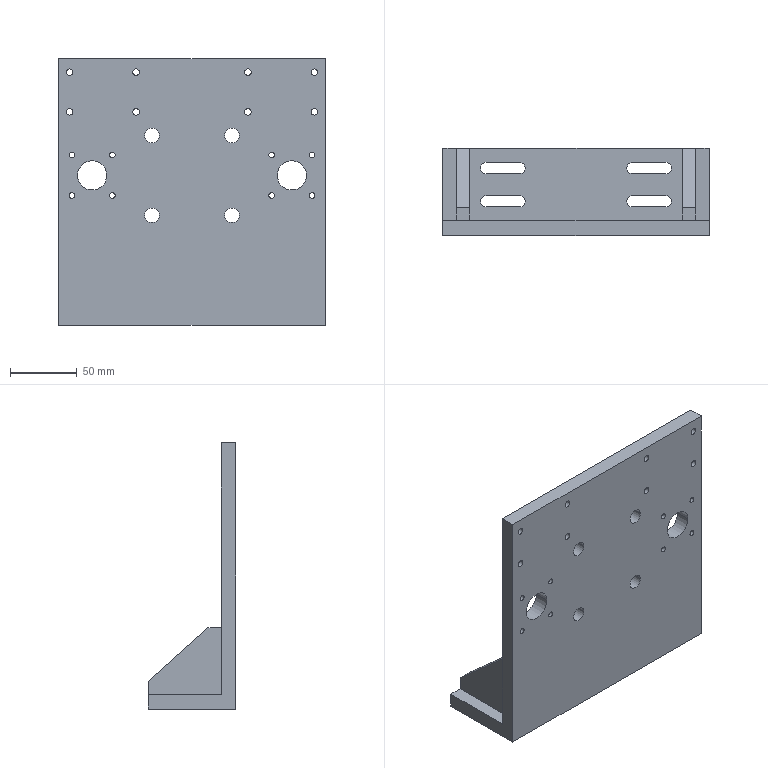Component | SolidWorks | YS01-053FixedBracket2-1 | 1 solid | 78 faces | box 200 x 66 x 200 mm | volume 570662 mm3 | cylinder 52 | plane 26 | commonest cylinder face diameters 5 x16 4.2 x16 11 x8 8.5 x8 22 x4
build123d program:
from build123d import *

# Parameters (mm, degrees)
SKETCH1_W                      = 200
SKETCH1_H                      = 200
BOSS_EXTRUDE1_DEPTH            = 11
SKETCH2_R                      = 11
CUT_EXTRUDE1_DEPTH             = 151.921
M5_TAPPED_HOLE1_AT_2_COUNT     = 2
M5_TAPPED_HOLE1_AT_2_PITCH     = 30.406
M5_TAPPED_HOLE1_AT_3_COUNT     = 2
M5_TAPPED_HOLE1_AT_3_PITCH     = 30.406
M5_TAPPED_HOLE1_AT_4_COUNT     = 2
M5_TAPPED_HOLE1_AT_4_PITCH     = 43
F_11_0_11_DIAMETER_HOLE2_D     = 11
F_11_0_11_DIAMETER_HOLE2_DEPTH = 14
F_11_0_11_DIAMETER_HOLE2_TIP   = 3.175
SKETCH7_W                      = 200
SKETCH7_H                      = 11
BOSS_EXTRUDE2_DEPTH            = 55
BOSS_EXTRUDE3_DEPTH            = 10
M6_TAPPED_HOLE1_AT_2_COUNT     = 2
M6_TAPPED_HOLE1_AT_2_PITCH     = 29.8
M6_TAPPED_HOLE1_AT_3_COUNT     = 2
M6_TAPPED_HOLE1_AT_3_PITCH     = 50
M6_TAPPED_HOLE1_AT_4_COUNT     = 2
M6_TAPPED_HOLE1_AT_4_PITCH     = 58.207
CUT_EXTRUDE2_DEPTH             = 224.779


with BuildPart() as part:
    # Sketch1 → Boss-Extrude1 (new body)
    with BuildSketch(Plane.XY):
        with Locations((0, -12.5)):
            Rectangle(SKETCH1_W, SKETCH1_H)
    extrude(amount=BOSS_EXTRUDE1_DEPTH)

    # Sketch2 → Cut-Extrude1 (cut, through all)
    with BuildSketch(Plane.XY.offset(11)):
        with Locations((75, 0)):
            Circle(SKETCH2_R)
        with Locations((-75, 0)):
            Circle(SKETCH2_R)
    extrude(amount=-CUT_EXTRUDE1_DEPTH, mode=Mode.SUBTRACT)

    # Sketch3 → M5 Tapped Hole1 (revolve, cut)
    with BuildSketch(Plane(origin=(90.203, 15.203, 0), x_dir=(0, 1, 0), z_dir=(1, 0, 0))):
        Polygon((0, 0), (0, 13.662), (2.1, 12.4), (2.1, 0), align=None)
    m5_tapped_hole1 = revolve(axis=Axis((90.203, 15.203, -6.35), (0, 0, 1)), mode=Mode.SUBTRACT)

    # M5 Tapped Hole1 at 2: M5 Tapped Hole1 ×2
    with Locations(*[(0, -i * M5_TAPPED_HOLE1_AT_2_PITCH, 0) for i in range(1, M5_TAPPED_HOLE1_AT_2_COUNT)]):
        add(m5_tapped_hole1, mode=Mode.SUBTRACT)

    # M5 Tapped Hole1 at 3: M5 Tapped Hole1 ×2
    with Locations(*[(-i * M5_TAPPED_HOLE1_AT_3_PITCH, 0, 0) for i in range(1, M5_TAPPED_HOLE1_AT_3_COUNT)]):
        add(m5_tapped_hole1, mode=Mode.SUBTRACT)

    # M5 Tapped Hole1 at 4: M5 Tapped Hole1 ×2
    with Locations(*[Vector(-0.7071, -0.7071, 0) * (i * M5_TAPPED_HOLE1_AT_4_PITCH) for i in range(1, M5_TAPPED_HOLE1_AT_4_COUNT)]):
        add(m5_tapped_hole1, mode=Mode.SUBTRACT)

    # Mirror1: M5 Tapped Hole1 across plane
    add(m5_tapped_hole1.mirror(Plane(origin=(0, 0, 0), x_dir=(0, 0, 1), z_dir=(1, 0, 0))), mode=Mode.SUBTRACT)

    # Mirror1 copy 1 sketch → Mirror1 copy 1 (revolve, cut)
    with BuildSketch(Plane(origin=(-90.203, -15.203, 0), x_dir=(0, 1, 0), z_dir=(-1, 0, 0))):
        Polygon((0, 0), (0, -13.662), (2.1, -12.4), (2.1, 0), align=None)
    revolve(axis=Axis((-90.203, -15.203, -6.35), (0, 0, -1)), mode=Mode.SUBTRACT)

    # Mirror1 copy 2 sketch → Mirror1 copy 2 (revolve, cut)
    with BuildSketch(Plane(origin=(-59.797, 15.203, 0), x_dir=(0, 1, 0), z_dir=(-1, 0, 0))):
        Polygon((0, 0), (0, -13.662), (2.1, -12.4), (2.1, 0), align=None)
    revolve(axis=Axis((-59.797, 15.203, -6.35), (0, 0, -1)), mode=Mode.SUBTRACT)

    # Mirror1 copy 3 sketch → Mirror1 copy 3 (revolve, cut)
    with BuildSketch(Plane(origin=(-59.797, -15.203, 0), x_dir=(0, 1, 0), z_dir=(-1, 0, 0))):
        Polygon((0, 0), (0, -13.662), (2.1, -12.4), (2.1, 0), align=None)
    revolve(axis=Axis((-59.797, -15.203, -6.35), (0, 0, -1)), mode=Mode.SUBTRACT)

    # 11.0 _11_ Diameter Hole2
    with Locations(Plane.XY.offset(11)):
        with Locations((30, -30), (-30, -30), (-30, 30), (30, 30)):
            Hole(F_11_0_11_DIAMETER_HOLE2_D / 2, depth=F_11_0_11_DIAMETER_HOLE2_DEPTH)
            with Locations((0, 0, -(F_11_0_11_DIAMETER_HOLE2_DEPTH + F_11_0_11_DIAMETER_HOLE2_TIP / 2))):  # 120° drill point
                Cone(0, F_11_0_11_DIAMETER_HOLE2_D / 2, F_11_0_11_DIAMETER_HOLE2_TIP, mode=Mode.SUBTRACT)

    # Sketch7 → Boss-Extrude2 (add)
    with BuildSketch(Plane.XY.offset(11)):
        with Locations((0, -107)):
            Rectangle(SKETCH7_W, SKETCH7_H)
    extrude(amount=BOSS_EXTRUDE2_DEPTH)

    # Sketch8 → Boss-Extrude3 (add)
    with BuildSketch(Plane.ZY.offset(90)):
        Polygon((11, -51.5), (21, -51.5), (66, -91.5), (66, -101.5), (11, -101.5), align=None)
    boss_extrude3 = extrude(amount=-BOSS_EXTRUDE3_DEPTH)

    # Sketch9 → M6 Tapped Hole1 (revolve, cut)
    with BuildSketch(Plane(origin=(-92, 77.5, 11), x_dir=(0, -1, 0), z_dir=(1, 0, 0))):
        Polygon((0, 0), (0, 16.502), (2.5, 15), (2.5, 0), align=None)
    m6_tapped_hole1 = revolve(axis=Axis((-92, 77.5, 17.35), (0, 0, -1)), mode=Mode.SUBTRACT)

    # M6 Tapped Hole1 at 2: M6 Tapped Hole1 ×2
    with Locations(*[(0, -i * M6_TAPPED_HOLE1_AT_2_PITCH, 0) for i in range(1, M6_TAPPED_HOLE1_AT_2_COUNT)]):
        add(m6_tapped_hole1, mode=Mode.SUBTRACT)

    # M6 Tapped Hole1 at 3: M6 Tapped Hole1 ×2
    with Locations(*[(i * M6_TAPPED_HOLE1_AT_3_PITCH, 0, 0) for i in range(1, M6_TAPPED_HOLE1_AT_3_COUNT)]):
        add(m6_tapped_hole1, mode=Mode.SUBTRACT)

    # M6 Tapped Hole1 at 4: M6 Tapped Hole1 ×2
    with Locations(*[Vector(0.859, -0.512, 0) * (i * M6_TAPPED_HOLE1_AT_4_PITCH) for i in range(1, M6_TAPPED_HOLE1_AT_4_COUNT)]):
        add(m6_tapped_hole1, mode=Mode.SUBTRACT)

    # Mirror2: Boss-Extrude3, M6 Tapped Hole1 across plane
    add(boss_extrude3.mirror(Plane.ZY))
    add(m6_tapped_hole1.mirror(Plane.ZY), mode=Mode.SUBTRACT)

    # Mirror2 copy 1 sketch → Mirror2 copy 1 (revolve, cut)
    with BuildSketch(Plane(origin=(92, 47.7, 11), x_dir=(0, -1, 0), z_dir=(-1, 0, 0))):
        Polygon((0, 0), (0, -16.502), (2.5, -15), (2.5, 0), align=None)
    revolve(axis=Axis((92, 47.7, 17.35), (0, 0, 1)), mode=Mode.SUBTRACT)

    # Mirror2 copy 2 sketch → Mirror2 copy 2 (revolve, cut)
    with BuildSketch(Plane(origin=(42, 77.5, 11), x_dir=(0, -1, 0), z_dir=(-1, 0, 0))):
        Polygon((0, 0), (0, -16.502), (2.5, -15), (2.5, 0), align=None)
    revolve(axis=Axis((42, 77.5, 17.35), (0, 0, 1)), mode=Mode.SUBTRACT)

    # Mirror2 copy 3 sketch → Mirror2 copy 3 (revolve, cut)
    with BuildSketch(Plane(origin=(42, 47.7, 11), x_dir=(0, -1, 0), z_dir=(-1, 0, 0))):
        Polygon((0, 0), (0, -16.502), (2.5, -15), (2.5, 0), align=None)
    revolve(axis=Axis((42, 47.7, 17.35), (0, 0, 1)), mode=Mode.SUBTRACT)

    # Sketch11 → Cut-Extrude2 (cut, through all)
    with BuildSketch(Plane(origin=(0, -101.5, 0), x_dir=(1, 0, 0), z_dir=(0, 1, 0))):
        with BuildLine():
            Line((-67.5, -21.75), (-42.5, -21.75))
            ThreePointArc((-42.5, -21.75), (-38.25, -26), (-42.5, -30.25))
            Line((-42.5, -30.25), (-67.5, -30.25))
            ThreePointArc((-67.5, -30.25), (-71.75, -26), (-67.5, -21.75))
        make_face()
        with BuildLine():
            Line((-67.5, -46.75), (-42.5, -46.75))
            ThreePointArc((-42.5, -46.75), (-38.25, -51), (-42.5, -55.25))
            Line((-42.5, -55.25), (-67.5, -55.25))
            ThreePointArc((-67.5, -55.25), (-71.75, -51), (-67.5, -46.75))
        make_face()
    cut_extrude2 = extrude(amount=-CUT_EXTRUDE2_DEPTH, mode=Mode.SUBTRACT)

    # Mirror3: Cut-Extrude2 across plane
    add(cut_extrude2.mirror(Plane.ZY), mode=Mode.SUBTRACT)


solid = part.part

# Placed as in the assembly
solid = solid.moved(Location((-566.612, -154.873, 2398.4), (-90, 0, 180)))